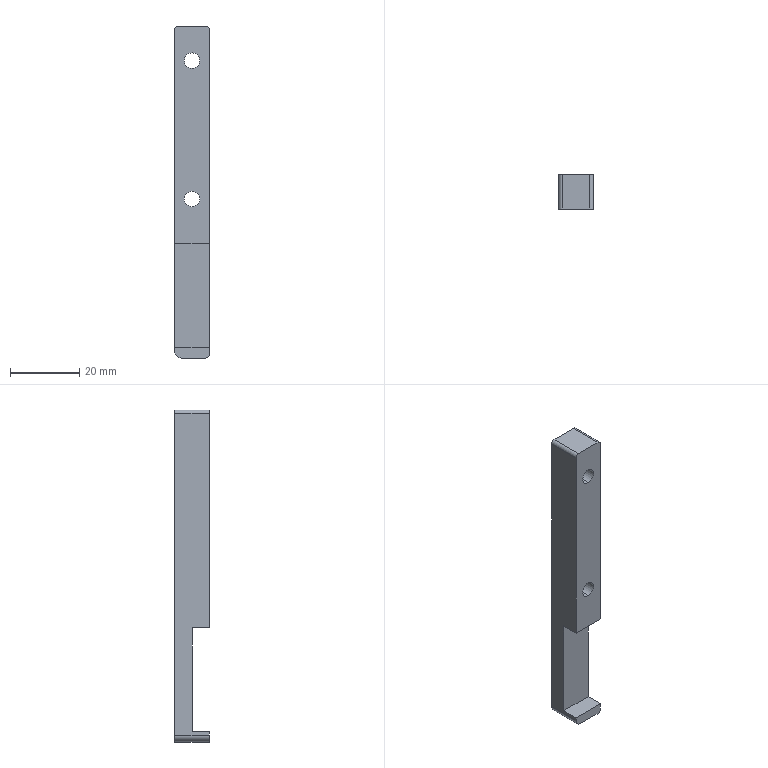Component | SolidWorks | SecondGenerationFour-sidedLabelingFeedingLimitPlate-1 | 1 solid | 24 faces | box 10 x 10 x 96 mm | volume 7451 mm3 | cylinder 12 | plane 12 | commonest cylinder face diameters 8 x4 4.5 x4 2 x3 4 x1
build123d program:
from build123d import *

# Parameters (mm, degrees)
SKETCH1_W                                            = 96
SKETCH1_H                                            = 10
BOSS_EXTRUDE1_DEPTH                                  = 10
HOLE_SIZE_ACCORDING_TO_THE_TYPE_OF_HEXAG_D           = 4.5
HOLE_SIZE_ACCORDING_TO_THE_TYPE_OF_HEXAG_CBORE_D     = 8
HOLE_SIZE_ACCORDING_TO_THE_TYPE_OF_HEXAG_CBORE_DEPTH = 4.6
SKETCH4_W                                            = 30
SKETCH4_H                                            = 5
CUT_EXTRUDE1_DEPTH                                   = 68.974
FILLET1_R                                            = 1
FILLET2_R                                            = 2


with BuildPart() as part:
    # Sketch1 → Boss-Extrude1 (new body)
    with BuildSketch(Plane.XY):
        with Locations((18.487, -24.142)):
            Rectangle(SKETCH1_W, SKETCH1_H)
    extrude(amount=BOSS_EXTRUDE1_DEPTH)

    # Hole Size according to the type of Hexag (through all)
    with Locations(Plane.XY.offset(10)):
        with Locations((-19.513, -24.142), (20.487, -24.142)):
            CounterBoreHole(HOLE_SIZE_ACCORDING_TO_THE_TYPE_OF_HEXAG_D / 2, HOLE_SIZE_ACCORDING_TO_THE_TYPE_OF_HEXAG_CBORE_D / 2, HOLE_SIZE_ACCORDING_TO_THE_TYPE_OF_HEXAG_CBORE_DEPTH)

    # Sketch4 → Cut-Extrude1 (cut, through all)
    with BuildSketch(Plane.XZ.offset(29.142)):
        with Locations((48.487, 2.5)):
            Rectangle(SKETCH4_W, SKETCH4_H)
    extrude(amount=-CUT_EXTRUDE1_DEPTH, mode=Mode.SUBTRACT)

    # Fillet1
    fillet1_edges = [part.edges().sort_by_distance(p)[0] for p in [
        (-29.513, -19.142, 5),
        (66.487, -29.142, 5),
        (-29.513, -29.142, 5),
    ]]
    fillet(fillet1_edges, radius=FILLET1_R)

    # Fillet2
    fillet2_edges = [part.edges().sort_by_distance(p)[0] for p in [
        (66.487, -19.142, 5),
    ]]
    fillet(fillet2_edges, radius=FILLET2_R)


solid = part.part

# Placed as in the assembly
solid = solid.moved(Location((-99.168, 41.863, -153.513), (-90, 0, 90)))
STEP:
#1=CARTESIAN_POINT('',(-2.954,1.861,-5.118));
#2=VERTEX_POINT('',#1);
#3=CARTESIAN_POINT('',(-2.954,1.861,-5.433));
#4=VERTEX_POINT('',#3);
#5=CARTESIAN_POINT('',(-2.954,1.861,-5.276));
#6=DIRECTION('',(0.,1.,0.));
#7=DIRECTION('',(0.,0.,-1.));
#8=AXIS2_PLACEMENT_3D('',#5,#6,#7);
#9=CIRCLE('',#8,0.1575);
#10=EDGE_CURVE('',#2,#4,#9,.T.);
#11=ORIENTED_EDGE('',*,*,#10,.F.);
#12=CARTESIAN_POINT('',(-2.954,2.042,-5.118));
#13=VERTEX_POINT('',#12);
#14=CARTESIAN_POINT('',(-2.954,2.042,-5.118));
#15=DIRECTION('',(0.,1.,0.));
#16=VECTOR('',#15,39.37);
#17=LINE('',#14,#16);
#18=EDGE_CURVE('',#2,#13,#17,.T.);
#19=ORIENTED_EDGE('',*,*,#18,.T.);
#20=CARTESIAN_POINT('',(-2.954,2.042,-5.433));
#21=VERTEX_POINT('',#20);
#22=CARTESIAN_POINT('',(-2.954,2.042,-5.276));
#23=DIRECTION('',(0.,1.,0.));
#24=DIRECTION('',(0.,0.,-1.));
#25=AXIS2_PLACEMENT_3D('',#22,#23,#24);
#26=CIRCLE('',#25,0.1575);
#27=EDGE_CURVE('',#13,#21,#26,.T.);
#28=ORIENTED_EDGE('',*,*,#27,.T.);
#29=CARTESIAN_POINT('',(-2.954,2.042,-5.433));
#30=DIRECTION('',(0.,1.,0.));
#31=VECTOR('',#30,39.37);
#32=LINE('',#29,#31);
#33=EDGE_CURVE('',#4,#21,#32,.T.);
#34=ORIENTED_EDGE('',*,*,#33,.F.);
#35=EDGE_LOOP('',(#11,#19,#28,#34));
#36=FACE_OUTER_BOUND('',#35,.T.);
#37=CARTESIAN_POINT('',(-2.954,2.042,-5.276));
#38=DIRECTION('',(0.,1.,0.));
#39=DIRECTION('',(0.,0.,-1.));
#40=AXIS2_PLACEMENT_3D('',#37,#38,#39);
#41=CYLINDRICAL_SURFACE('',#40,0.1575);
#42=ADVANCED_FACE('',(#36),#41,.F.);
#43=CARTESIAN_POINT('',(-2.954,1.648,-5.187));
#44=VERTEX_POINT('',#43);
#45=CARTESIAN_POINT('',(-2.954,1.648,-5.364));
#46=VERTEX_POINT('',#45);
#47=CARTESIAN_POINT('',(-2.954,1.648,-5.276));
#48=DIRECTION('',(0.,1.,0.));
#49=DIRECTION('',(0.,0.,-1.));
#50=AXIS2_PLACEMENT_3D('',#47,#48,#49);
#51=CIRCLE('',#50,0.08858);
#52=EDGE_CURVE('',#44,#46,#51,.T.);
#53=ORIENTED_EDGE('',*,*,#52,.F.);
#54=CARTESIAN_POINT('',(-2.954,1.861,-5.187));
#55=VERTEX_POINT('',#54);
#56=CARTESIAN_POINT('',(-2.954,2.042,-5.187));
#57=DIRECTION('',(0.,1.,0.));
#58=VECTOR('',#57,39.37);
#59=LINE('',#56,#58);
#60=EDGE_CURVE('',#44,#55,#59,.T.);
#61=ORIENTED_EDGE('',*,*,#60,.T.);
#62=CARTESIAN_POINT('',(-2.954,1.861,-5.364));
#63=VERTEX_POINT('',#62);
#64=CARTESIAN_POINT('',(-2.954,1.861,-5.276));
#65=DIRECTION('',(0.,1.,0.));
#66=DIRECTION('',(0.,0.,-1.));
#67=AXIS2_PLACEMENT_3D('',#64,#65,#66);
#68=CIRCLE('',#67,0.08858);
#69=EDGE_CURVE('',#55,#63,#68,.T.);
#70=ORIENTED_EDGE('',*,*,#69,.T.);
#71=CARTESIAN_POINT('',(-2.954,2.042,-5.364));
#72=DIRECTION('',(0.,1.,0.));
#73=VECTOR('',#72,39.37);
#74=LINE('',#71,#73);
#75=EDGE_CURVE('',#46,#63,#74,.T.);
#76=ORIENTED_EDGE('',*,*,#75,.F.);
#77=EDGE_LOOP('',(#53,#61,#70,#76));
#78=FACE_OUTER_BOUND('',#77,.T.);
#79=CARTESIAN_POINT('',(-2.954,2.042,-5.276));
#80=DIRECTION('',(0.,1.,0.));
#81=DIRECTION('',(0.,0.,-1.));
#82=AXIS2_PLACEMENT_3D('',#79,#80,#81);
#83=CYLINDRICAL_SURFACE('',#82,0.08858);
#84=ADVANCED_FACE('',(#78),#83,.F.);
#85=CARTESIAN_POINT('',(-2.954,1.861,-6.693));
#86=VERTEX_POINT('',#85);
#87=CARTESIAN_POINT('',(-2.954,1.861,-7.008));
#88=VERTEX_POINT('',#87);
#89=CARTESIAN_POINT('',(-2.954,1.861,-6.85));
#90=DIRECTION('',(0.,1.,0.));
#91=DIRECTION('',(0.,0.,-1.));
#92=AXIS2_PLACEMENT_3D('',#89,#90,#91);
#93=CIRCLE('',#92,0.1575);
#94=EDGE_CURVE('',#86,#88,#93,.T.);
#95=ORIENTED_EDGE('',*,*,#94,.F.);
#96=CARTESIAN_POINT('',(-2.954,2.042,-6.693));
#97=VERTEX_POINT('',#96);
#98=CARTESIAN_POINT('',(-2.954,2.042,-6.693));
#99=DIRECTION('',(0.,1.,0.));
#100=VECTOR('',#99,39.37);
#101=LINE('',#98,#100);
#102=EDGE_CURVE('',#86,#97,#101,.T.);
#103=ORIENTED_EDGE('',*,*,#102,.T.);
#104=CARTESIAN_POINT('',(-2.954,2.042,-7.008));
#105=VERTEX_POINT('',#104);
#106=CARTESIAN_POINT('',(-2.954,2.042,-6.85));
#107=DIRECTION('',(0.,1.,0.));
#108=DIRECTION('',(0.,0.,-1.));
#109=AXIS2_PLACEMENT_3D('',#106,#107,#108);
#110=CIRCLE('',#109,0.1575);
#111=EDGE_CURVE('',#97,#105,#110,.T.);
#112=ORIENTED_EDGE('',*,*,#111,.T.);
#113=CARTESIAN_POINT('',(-2.954,2.042,-7.008));
#114=DIRECTION('',(0.,1.,0.));
#115=VECTOR('',#114,39.37);
#116=LINE('',#113,#115);
#117=EDGE_CURVE('',#88,#105,#116,.T.);
#118=ORIENTED_EDGE('',*,*,#117,.F.);
#119=EDGE_LOOP('',(#95,#103,#112,#118));
#120=FACE_OUTER_BOUND('',#119,.T.);
#121=CARTESIAN_POINT('',(-2.954,2.042,-6.85));
#122=DIRECTION('',(0.,1.,0.));
#123=DIRECTION('',(0.,0.,-1.));
#124=AXIS2_PLACEMENT_3D('',#121,#122,#123);
#125=CYLINDRICAL_SURFACE('',#124,0.1575);
#126=ADVANCED_FACE('',(#120),#125,.F.);
#127=CARTESIAN_POINT('',(-2.954,1.648,-6.762));
#128=VERTEX_POINT('',#127);
#129=CARTESIAN_POINT('',(-2.954,1.648,-6.939));
#130=VERTEX_POINT('',#129);
#131=CARTESIAN_POINT('',(-2.954,1.648,-6.85));
#132=DIRECTION('',(0.,1.,0.));
#133=DIRECTION('',(0.,0.,-1.));
#134=AXIS2_PLACEMENT_3D('',#131,#132,#133);
#135=CIRCLE('',#134,0.08858);
#136=EDGE_CURVE('',#128,#130,#135,.T.);
#137=ORIENTED_EDGE('',*,*,#136,.F.);
#138=CARTESIAN_POINT('',(-2.954,1.861,-6.762));
#139=VERTEX_POINT('',#138);
#140=CARTESIAN_POINT('',(-2.954,2.042,-6.762));
#141=DIRECTION('',(0.,1.,0.));
#142=VECTOR('',#141,39.37);
#143=LINE('',#140,#142);
#144=EDGE_CURVE('',#128,#139,#143,.T.);
#145=ORIENTED_EDGE('',*,*,#144,.T.);
#146=CARTESIAN_POINT('',(-2.954,1.861,-6.939));
#147=VERTEX_POINT('',#146);
#148=CARTESIAN_POINT('',(-2.954,1.861,-6.85));
#149=DIRECTION('',(0.,1.,0.));
#150=DIRECTION('',(0.,0.,-1.));
#151=AXIS2_PLACEMENT_3D('',#148,#149,#150);
#152=CIRCLE('',#151,0.08858);
#153=EDGE_CURVE('',#139,#147,#152,.T.);
#154=ORIENTED_EDGE('',*,*,#153,.T.);
#155=CARTESIAN_POINT('',(-2.954,2.042,-6.939));
#156=DIRECTION('',(0.,1.,0.));
#157=VECTOR('',#156,39.37);
#158=LINE('',#155,#157);
#159=EDGE_CURVE('',#130,#147,#158,.T.);
#160=ORIENTED_EDGE('',*,*,#159,.F.);
#161=EDGE_LOOP('',(#137,#145,#154,#160));
#162=FACE_OUTER_BOUND('',#161,.T.);
#163=CARTESIAN_POINT('',(-2.954,2.042,-6.85));
#164=DIRECTION('',(0.,1.,0.));
#165=DIRECTION('',(0.,0.,-1.));
#166=AXIS2_PLACEMENT_3D('',#163,#164,#165);
#167=CYLINDRICAL_SURFACE('',#166,0.08858);
#168=ADVANCED_FACE('',(#162),#167,.F.);
#169=CARTESIAN_POINT('',(-2.954,1.648,-6.85));
#170=DIRECTION('',(0.,1.,0.));
#171=DIRECTION('',(0.,0.,-1.));
#172=AXIS2_PLACEMENT_3D('',#169,#170,#171);
#173=CIRCLE('',#172,0.08858);
#174=EDGE_CURVE('',#130,#128,#173,.T.);
#175=ORIENTED_EDGE('',*,*,#174,.T.);
#176=ORIENTED_EDGE('',*,*,#136,.T.);
#177=EDGE_LOOP('',(#175,#176));
#178=FACE_BOUND('',#177,.T.);
#179=CARTESIAN_POINT('',(-2.954,1.648,-5.276));
#180=DIRECTION('',(0.,1.,0.));
#181=DIRECTION('',(0.,0.,-1.));
#182=AXIS2_PLACEMENT_3D('',#179,#180,#181);
#183=CIRCLE('',#182,0.08858);
#184=EDGE_CURVE('',#46,#44,#183,.T.);
#185=ORIENTED_EDGE('',*,*,#184,.T.);
#186=ORIENTED_EDGE('',*,*,#52,.T.);
#187=EDGE_LOOP('',(#185,#186));
#188=FACE_BOUND('',#187,.T.);
#189=CARTESIAN_POINT('',(-3.111,1.648,-4.882));
#190=VERTEX_POINT('',#189);
#191=CARTESIAN_POINT('',(-2.796,1.648,-4.882));
#192=VERTEX_POINT('',#191);
#193=CARTESIAN_POINT('',(-3.151,1.648,-4.882));
#194=DIRECTION('',(1.,0.,0.));
#195=VECTOR('',#194,39.37);
#196=LINE('',#193,#195);
#197=EDGE_CURVE('',#190,#192,#196,.T.);
#198=ORIENTED_EDGE('',*,*,#197,.F.);
#199=CARTESIAN_POINT('',(-3.151,1.648,-4.921));
#200=VERTEX_POINT('',#199);
#201=CARTESIAN_POINT('',(-3.111,1.648,-4.921));
#202=DIRECTION('',(0.,-1.,0.));
#203=DIRECTION('',(0.,0.,-1.));
#204=AXIS2_PLACEMENT_3D('',#201,#202,#203);
#205=CIRCLE('',#204,0.03937);
#206=EDGE_CURVE('',#190,#200,#205,.T.);
#207=ORIENTED_EDGE('',*,*,#206,.T.);
#208=CARTESIAN_POINT('',(-3.151,1.648,-7.362));
#209=VERTEX_POINT('',#208);
#210=CARTESIAN_POINT('',(-3.151,1.648,-4.882));
#211=DIRECTION('',(0.,0.,1.));
#212=VECTOR('',#211,39.37);
#213=LINE('',#210,#212);
#214=EDGE_CURVE('',#209,#200,#213,.T.);
#215=ORIENTED_EDGE('',*,*,#214,.F.);
#216=CARTESIAN_POINT('',(-2.757,1.648,-7.362));
#217=VERTEX_POINT('',#216);
#218=CARTESIAN_POINT('',(-3.151,1.648,-7.362));
#219=DIRECTION('',(1.,0.,0.));
#220=VECTOR('',#219,39.37);
#221=LINE('',#218,#220);
#222=EDGE_CURVE('',#209,#217,#221,.T.);
#223=ORIENTED_EDGE('',*,*,#222,.T.);
#224=CARTESIAN_POINT('',(-2.757,1.648,-4.921));
#225=VERTEX_POINT('',#224);
#226=CARTESIAN_POINT('',(-2.757,1.648,-4.882));
#227=DIRECTION('',(0.,0.,-1.));
#228=VECTOR('',#227,39.37);
#229=LINE('',#226,#228);
#230=EDGE_CURVE('',#225,#217,#229,.T.);
#231=ORIENTED_EDGE('',*,*,#230,.F.);
#232=CARTESIAN_POINT('',(-2.796,1.648,-4.921));
#233=DIRECTION('',(0.,-1.,0.));
#234=DIRECTION('',(0.,0.,-1.));
#235=AXIS2_PLACEMENT_3D('',#232,#233,#234);
#236=CIRCLE('',#235,0.03937);
#237=EDGE_CURVE('',#225,#192,#236,.T.);
#238=ORIENTED_EDGE('',*,*,#237,.T.);
#239=EDGE_LOOP('',(#198,#207,#215,#223,#231,#238));
#240=FACE_OUTER_BOUND('',#239,.T.);
#241=CARTESIAN_POINT('',(-2.757,1.648,-4.882));
#242=DIRECTION('',(0.,1.,0.));
#243=DIRECTION('',(0.,0.,-1.));
#244=AXIS2_PLACEMENT_3D('',#241,#242,#243);
#245=PLANE('',#244);
#246=ADVANCED_FACE('',(#178,#188,#240),#245,.F.);
#247=CARTESIAN_POINT('',(-3.111,2.042,-4.882));
#248=VERTEX_POINT('',#247);
#249=CARTESIAN_POINT('',(-2.796,2.042,-4.882));
#250=VERTEX_POINT('',#249);
#251=CARTESIAN_POINT('',(-3.151,2.042,-4.882));
#252=DIRECTION('',(1.,0.,0.));
#253=VECTOR('',#252,39.37);
#254=LINE('',#251,#253);
#255=EDGE_CURVE('',#248,#250,#254,.T.);
#256=ORIENTED_EDGE('',*,*,#255,.F.);
#257=CARTESIAN_POINT('',(-3.111,2.042,-4.882));
#258=DIRECTION('',(0.,-1.,0.));
#259=VECTOR('',#258,39.37);
#260=LINE('',#257,#259);
#261=EDGE_CURVE('',#248,#190,#260,.T.);
#262=ORIENTED_EDGE('',*,*,#261,.T.);
#263=ORIENTED_EDGE('',*,*,#197,.T.);
#264=CARTESIAN_POINT('',(-2.796,2.042,-4.882));
#265=DIRECTION('',(0.,1.,0.));
#266=VECTOR('',#265,39.37);
#267=LINE('',#264,#266);
#268=EDGE_CURVE('',#192,#250,#267,.T.);
#269=ORIENTED_EDGE('',*,*,#268,.T.);
#270=EDGE_LOOP('',(#256,#262,#263,#269));
#271=FACE_OUTER_BOUND('',#270,.T.);
#272=CARTESIAN_POINT('',(-3.151,2.042,-4.882));
#273=DIRECTION('',(0.,0.,-1.));
#274=DIRECTION('',(0.,-1.,0.));
#275=AXIS2_PLACEMENT_3D('',#272,#273,#274);
#276=PLANE('',#275);
#277=ADVANCED_FACE('',(#271),#276,.F.);
#278=CARTESIAN_POINT('',(-2.757,1.648,-8.543));
#279=VERTEX_POINT('',#278);
#280=CARTESIAN_POINT('',(-2.757,1.648,-8.622));
#281=VERTEX_POINT('',#280);
#282=CARTESIAN_POINT('',(-2.757,1.648,-4.882));
#283=DIRECTION('',(0.,0.,-1.));
#284=VECTOR('',#283,39.37);
#285=LINE('',#282,#284);
#286=EDGE_CURVE('',#279,#281,#285,.T.);
#287=ORIENTED_EDGE('',*,*,#286,.T.);
#288=CARTESIAN_POINT('',(-2.757,2.042,-8.622));
#289=VERTEX_POINT('',#288);
#290=CARTESIAN_POINT('',(-2.757,2.042,-8.622));
#291=DIRECTION('',(0.,1.,0.));
#292=VECTOR('',#291,39.37);
#293=LINE('',#290,#292);
#294=EDGE_CURVE('',#281,#289,#293,.T.);
#295=ORIENTED_EDGE('',*,*,#294,.T.);
#296=CARTESIAN_POINT('',(-2.757,2.042,-4.921));
#297=VERTEX_POINT('',#296);
#298=CARTESIAN_POINT('',(-2.757,2.042,-4.882));
#299=DIRECTION('',(0.,0.,-1.));
#300=VECTOR('',#299,39.37);
#301=LINE('',#298,#300);
#302=EDGE_CURVE('',#297,#289,#301,.T.);
#303=ORIENTED_EDGE('',*,*,#302,.F.);
#304=CARTESIAN_POINT('',(-2.757,2.042,-4.921));
#305=DIRECTION('',(0.,-1.,0.));
#306=VECTOR('',#305,39.37);
#307=LINE('',#304,#306);
#308=EDGE_CURVE('',#297,#225,#307,.T.);
#309=ORIENTED_EDGE('',*,*,#308,.T.);
#310=ORIENTED_EDGE('',*,*,#230,.T.);
#311=CARTESIAN_POINT('',(-2.757,1.845,-7.362));
#312=VERTEX_POINT('',#311);
#313=CARTESIAN_POINT('',(-2.757,1.845,-7.362));
#314=DIRECTION('',(0.,-1.,0.));
#315=VECTOR('',#314,39.37);
#316=LINE('',#313,#315);
#317=EDGE_CURVE('',#312,#217,#316,.T.);
#318=ORIENTED_EDGE('',*,*,#317,.F.);
#319=CARTESIAN_POINT('',(-2.757,1.845,-8.543));
#320=VERTEX_POINT('',#319);
#321=CARTESIAN_POINT('',(-2.757,1.845,-7.362));
#322=DIRECTION('',(0.,0.,1.));
#323=VECTOR('',#322,39.37);
#324=LINE('',#321,#323);
#325=EDGE_CURVE('',#320,#312,#324,.T.);
#326=ORIENTED_EDGE('',*,*,#325,.F.);
#327=CARTESIAN_POINT('',(-2.757,1.845,-8.543));
#328=DIRECTION('',(0.,1.,0.));
#329=VECTOR('',#328,39.37);
#330=LINE('',#327,#329);
#331=EDGE_CURVE('',#279,#320,#330,.T.);
#332=ORIENTED_EDGE('',*,*,#331,.F.);
#333=EDGE_LOOP('',(#287,#295,#303,#309,#310,#318,#326,#332));
#334=FACE_OUTER_BOUND('',#333,.T.);
#335=CARTESIAN_POINT('',(-2.757,2.042,-4.882));
#336=DIRECTION('',(-1.,0.,0.));
#337=DIRECTION('',(0.,1.,0.));
#338=AXIS2_PLACEMENT_3D('',#335,#336,#337);
#339=PLANE('',#338);
#340=ADVANCED_FACE('',(#334),#339,.F.);
#341=CARTESIAN_POINT('',(-2.796,1.648,-8.661));
#342=VERTEX_POINT('',#341);
#343=CARTESIAN_POINT('',(-3.072,1.648,-8.661));
#344=VERTEX_POINT('',#343);
#345=CARTESIAN_POINT('',(-3.151,1.648,-8.661));
#346=DIRECTION('',(-1.,0.,0.));
#347=VECTOR('',#346,39.37);
#348=LINE('',#345,#347);
#349=EDGE_CURVE('',#342,#344,#348,.T.);
#350=ORIENTED_EDGE('',*,*,#349,.T.);
#351=CARTESIAN_POINT('',(-3.072,2.042,-8.661));
#352=VERTEX_POINT('',#351);
#353=CARTESIAN_POINT('',(-3.072,2.042,-8.661));
#354=DIRECTION('',(0.,1.,0.));
#355=VECTOR('',#354,39.37);
#356=LINE('',#353,#355);
#357=EDGE_CURVE('',#344,#352,#356,.T.);
#358=ORIENTED_EDGE('',*,*,#357,.T.);
#359=CARTESIAN_POINT('',(-2.796,2.042,-8.661));
#360=VERTEX_POINT('',#359);
#361=CARTESIAN_POINT('',(-3.151,2.042,-8.661));
#362=DIRECTION('',(-1.,0.,0.));
#363=VECTOR('',#362,39.37);
#364=LINE('',#361,#363);
#365=EDGE_CURVE('',#360,#352,#364,.T.);
#366=ORIENTED_EDGE('',*,*,#365,.F.);
#367=CARTESIAN_POINT('',(-2.796,2.042,-8.661));
#368=DIRECTION('',(0.,-1.,0.));
#369=VECTOR('',#368,39.37);
#370=LINE('',#367,#369);
#371=EDGE_CURVE('',#360,#342,#370,.T.);
#372=ORIENTED_EDGE('',*,*,#371,.T.);
#373=EDGE_LOOP('',(#350,#358,#366,#372));
#374=FACE_OUTER_BOUND('',#373,.T.);
#375=CARTESIAN_POINT('',(-3.151,2.042,-8.661));
#376=DIRECTION('',(0.,0.,1.));
#377=DIRECTION('',(0.,1.,0.));
#378=AXIS2_PLACEMENT_3D('',#375,#376,#377);
#379=PLANE('',#378);
#380=ADVANCED_FACE('',(#374),#379,.F.);
#381=CARTESIAN_POINT('',(-3.151,2.042,-8.583));
#382=VERTEX_POINT('',#381);
#383=CARTESIAN_POINT('',(-3.151,2.042,-4.921));
#384=VERTEX_POINT('',#383);
#385=CARTESIAN_POINT('',(-3.151,2.042,-4.882));
#386=DIRECTION('',(0.,0.,1.));
#387=VECTOR('',#386,39.37);
#388=LINE('',#385,#387);
#389=EDGE_CURVE('',#382,#384,#388,.T.);
#390=ORIENTED_EDGE('',*,*,#389,.F.);
#391=CARTESIAN_POINT('',(-3.151,1.648,-8.583));
#392=VERTEX_POINT('',#391);
#393=CARTESIAN_POINT('',(-3.151,2.042,-8.583));
#394=DIRECTION('',(0.,-1.,0.));
#395=VECTOR('',#394,39.37);
#396=LINE('',#393,#395);
#397=EDGE_CURVE('',#382,#392,#396,.T.);
#398=ORIENTED_EDGE('',*,*,#397,.T.);
#399=CARTESIAN_POINT('',(-3.151,1.648,-8.543));
#400=VERTEX_POINT('',#399);
#401=CARTESIAN_POINT('',(-3.151,1.648,-4.882));
#402=DIRECTION('',(0.,0.,1.));
#403=VECTOR('',#402,39.37);
#404=LINE('',#401,#403);
#405=EDGE_CURVE('',#392,#400,#404,.T.);
#406=ORIENTED_EDGE('',*,*,#405,.T.);
#407=CARTESIAN_POINT('',(-3.151,1.845,-8.543));
#408=VERTEX_POINT('',#407);
#409=CARTESIAN_POINT('',(-3.151,1.845,-8.543));
#410=DIRECTION('',(0.,1.,0.));
#411=VECTOR('',#410,39.37);
#412=LINE('',#409,#411);
#413=EDGE_CURVE('',#400,#408,#412,.T.);
#414=ORIENTED_EDGE('',*,*,#413,.T.);
#415=CARTESIAN_POINT('',(-3.151,1.845,-7.362));
#416=VERTEX_POINT('',#415);
#417=CARTESIAN_POINT('',(-3.151,1.845,-7.362));
#418=DIRECTION('',(0.,0.,1.));
#419=VECTOR('',#418,39.37);
#420=LINE('',#417,#419);
#421=EDGE_CURVE('',#408,#416,#420,.T.);
#422=ORIENTED_EDGE('',*,*,#421,.T.);
#423=CARTESIAN_POINT('',(-3.151,1.845,-7.362));
#424=DIRECTION('',(0.,-1.,0.));
#425=VECTOR('',#424,39.37);
#426=LINE('',#423,#425);
#427=EDGE_CURVE('',#416,#209,#426,.T.);
#428=ORIENTED_EDGE('',*,*,#427,.T.);
#429=ORIENTED_EDGE('',*,*,#214,.T.);
#430=CARTESIAN_POINT('',(-3.151,2.042,-4.921));
#431=DIRECTION('',(0.,1.,0.));
#432=VECTOR('',#431,39.37);
#433=LINE('',#430,#432);
#434=EDGE_CURVE('',#200,#384,#433,.T.);
#435=ORIENTED_EDGE('',*,*,#434,.T.);
#436=EDGE_LOOP('',(#390,#398,#406,#414,#422,#428,#429,#435));
#437=FACE_OUTER_BOUND('',#436,.T.);
#438=CARTESIAN_POINT('',(-3.151,2.042,-4.882));
#439=DIRECTION('',(1.,0.,0.));
#440=DIRECTION('',(0.,-1.,0.));
#441=AXIS2_PLACEMENT_3D('',#438,#439,#440);
#442=PLANE('',#441);
#443=ADVANCED_FACE('',(#437),#442,.F.);
#444=CARTESIAN_POINT('',(-2.954,2.042,-5.276));
#445=DIRECTION('',(0.,1.,0.));
#446=DIRECTION('',(0.,0.,-1.));
#447=AXIS2_PLACEMENT_3D('',#444,#445,#446);
#448=CIRCLE('',#447,0.1575);
#449=EDGE_CURVE('',#21,#13,#448,.T.);
#450=ORIENTED_EDGE('',*,*,#449,.F.);
#451=ORIENTED_EDGE('',*,*,#27,.F.);
#452=EDGE_LOOP('',(#450,#451));
#453=FACE_BOUND('',#452,.T.);
#454=CARTESIAN_POINT('',(-2.954,2.042,-6.85));
#455=DIRECTION('',(0.,1.,0.));
#456=DIRECTION('',(0.,0.,-1.));
#457=AXIS2_PLACEMENT_3D('',#454,#455,#456);
#458=CIRCLE('',#457,0.1575);
#459=EDGE_CURVE('',#105,#97,#458,.T.);
#460=ORIENTED_EDGE('',*,*,#459,.F.);
#461=ORIENTED_EDGE('',*,*,#111,.F.);
#462=EDGE_LOOP('',(#460,#461));
#463=FACE_BOUND('',#462,.T.);
#464=ORIENTED_EDGE('',*,*,#365,.T.);
#465=CARTESIAN_POINT('',(-3.072,2.042,-8.583));
#466=DIRECTION('',(0.,1.,0.));
#467=DIRECTION('',(0.,0.,-1.));
#468=AXIS2_PLACEMENT_3D('',#465,#466,#467);
#469=CIRCLE('',#468,0.07874);
#470=EDGE_CURVE('',#352,#382,#469,.T.);
#471=ORIENTED_EDGE('',*,*,#470,.T.);
#472=ORIENTED_EDGE('',*,*,#389,.T.);
#473=CARTESIAN_POINT('',(-3.111,2.042,-4.921));
#474=DIRECTION('',(0.,1.,0.));
#475=DIRECTION('',(0.,0.,-1.));
#476=AXIS2_PLACEMENT_3D('',#473,#474,#475);
#477=CIRCLE('',#476,0.03937);
#478=EDGE_CURVE('',#384,#248,#477,.T.);
#479=ORIENTED_EDGE('',*,*,#478,.T.);
#480=ORIENTED_EDGE('',*,*,#255,.T.);
#481=CARTESIAN_POINT('',(-2.796,2.042,-4.921));
#482=DIRECTION('',(0.,1.,0.));
#483=DIRECTION('',(0.,0.,-1.));
#484=AXIS2_PLACEMENT_3D('',#481,#482,#483);
#485=CIRCLE('',#484,0.03937);
#486=EDGE_CURVE('',#250,#297,#485,.T.);
#487=ORIENTED_EDGE('',*,*,#486,.T.);
#488=ORIENTED_EDGE('',*,*,#302,.T.);
#489=CARTESIAN_POINT('',(-2.796,2.042,-8.622));
#490=DIRECTION('',(0.,1.,0.));
#491=DIRECTION('',(0.,0.,-1.));
#492=AXIS2_PLACEMENT_3D('',#489,#490,#491);
#493=CIRCLE('',#492,0.03937);
#494=EDGE_CURVE('',#289,#360,#493,.T.);
#495=ORIENTED_EDGE('',*,*,#494,.T.);
#496=EDGE_LOOP('',(#464,#471,#472,#479,#480,#487,#488,#495));
#497=FACE_OUTER_BOUND('',#496,.T.);
#498=CARTESIAN_POINT('',(-2.757,2.042,-4.882));
#499=DIRECTION('',(0.,1.,0.));
#500=DIRECTION('',(0.,0.,-1.));
#501=AXIS2_PLACEMENT_3D('',#498,#499,#500);
#502=PLANE('',#501);
#503=ADVANCED_FACE('',(#453,#463,#497),#502,.T.);
#504=ORIENTED_EDGE('',*,*,#405,.F.);
#505=CARTESIAN_POINT('',(-3.072,1.648,-8.583));
#506=DIRECTION('',(0.,-1.,0.));
#507=DIRECTION('',(0.,0.,-1.));
#508=AXIS2_PLACEMENT_3D('',#505,#506,#507);
#509=CIRCLE('',#508,0.07874);
#510=EDGE_CURVE('',#392,#344,#509,.T.);
#511=ORIENTED_EDGE('',*,*,#510,.T.);
#512=ORIENTED_EDGE('',*,*,#349,.F.);
#513=CARTESIAN_POINT('',(-2.796,1.648,-8.622));
#514=DIRECTION('',(0.,-1.,0.));
#515=DIRECTION('',(0.,0.,-1.));
#516=AXIS2_PLACEMENT_3D('',#513,#514,#515);
#517=CIRCLE('',#516,0.03937);
#518=EDGE_CURVE('',#342,#281,#517,.T.);
#519=ORIENTED_EDGE('',*,*,#518,.T.);
#520=ORIENTED_EDGE('',*,*,#286,.F.);
#521=CARTESIAN_POINT('',(-3.151,1.648,-8.543));
#522=DIRECTION('',(1.,0.,0.));
#523=VECTOR('',#522,39.37);
#524=LINE('',#521,#523);
#525=EDGE_CURVE('',#400,#279,#524,.T.);
#526=ORIENTED_EDGE('',*,*,#525,.F.);
#527=EDGE_LOOP('',(#504,#511,#512,#519,#520,#526));
#528=FACE_OUTER_BOUND('',#527,.T.);
#529=CARTESIAN_POINT('',(-2.757,1.648,-4.882));
#530=DIRECTION('',(0.,1.,0.));
#531=DIRECTION('',(0.,0.,-1.));
#532=AXIS2_PLACEMENT_3D('',#529,#530,#531);
#533=PLANE('',#532);
#534=ADVANCED_FACE('',(#528),#533,.F.);
#535=ORIENTED_EDGE('',*,*,#144,.F.);
#536=ORIENTED_EDGE('',*,*,#174,.F.);
#537=ORIENTED_EDGE('',*,*,#159,.T.);
#538=CARTESIAN_POINT('',(-2.954,1.861,-6.85));
#539=DIRECTION('',(0.,1.,0.));
#540=DIRECTION('',(0.,0.,-1.));
#541=AXIS2_PLACEMENT_3D('',#538,#539,#540);
#542=CIRCLE('',#541,0.08858);
#543=EDGE_CURVE('',#147,#139,#542,.T.);
#544=ORIENTED_EDGE('',*,*,#543,.T.);
#545=EDGE_LOOP('',(#535,#536,#537,#544));
#546=FACE_OUTER_BOUND('',#545,.T.);
#547=CARTESIAN_POINT('',(-2.954,2.042,-6.85));
#548=DIRECTION('',(0.,1.,0.));
#549=DIRECTION('',(0.,0.,-1.));
#550=AXIS2_PLACEMENT_3D('',#547,#548,#549);
#551=CYLINDRICAL_SURFACE('',#550,0.08858);
#552=ADVANCED_FACE('',(#546),#551,.F.);
#553=ORIENTED_EDGE('',*,*,#543,.F.);
#554=ORIENTED_EDGE('',*,*,#153,.F.);
#555=EDGE_LOOP('',(#553,#554));
#556=FACE_BOUND('',#555,.T.);
#557=CARTESIAN_POINT('',(-2.954,1.861,-6.85));
#558=DIRECTION('',(0.,1.,0.));
#559=DIRECTION('',(0.,0.,-1.));
#560=AXIS2_PLACEMENT_3D('',#557,#558,#559);
#561=CIRCLE('',#560,0.1575);
#562=EDGE_CURVE('',#88,#86,#561,.T.);
#563=ORIENTED_EDGE('',*,*,#562,.T.);
#564=ORIENTED_EDGE('',*,*,#94,.T.);
#565=EDGE_LOOP('',(#563,#564));
#566=FACE_OUTER_BOUND('',#565,.T.);
#567=CARTESIAN_POINT('',(-2.954,1.861,-6.939));
#568=DIRECTION('',(0.,-1.,0.));
#569=DIRECTION('',(0.,0.,1.));
#570=AXIS2_PLACEMENT_3D('',#567,#568,#569);
#571=PLANE('',#570);
#572=ADVANCED_FACE('',(#556,#566),#571,.F.);
#573=ORIENTED_EDGE('',*,*,#102,.F.);
#574=ORIENTED_EDGE('',*,*,#562,.F.);
#575=ORIENTED_EDGE('',*,*,#117,.T.);
#576=ORIENTED_EDGE('',*,*,#459,.T.);
#577=EDGE_LOOP('',(#573,#574,#575,#576));
#578=FACE_OUTER_BOUND('',#577,.T.);
#579=CARTESIAN_POINT('',(-2.954,2.042,-6.85));
#580=DIRECTION('',(0.,1.,0.));
#581=DIRECTION('',(0.,0.,-1.));
#582=AXIS2_PLACEMENT_3D('',#579,#580,#581);
#583=CYLINDRICAL_SURFACE('',#582,0.1575);
#584=ADVANCED_FACE('',(#578),#583,.F.);
#585=ORIENTED_EDGE('',*,*,#60,.F.);
#586=ORIENTED_EDGE('',*,*,#184,.F.);
#587=ORIENTED_EDGE('',*,*,#75,.T.);
#588=CARTESIAN_POINT('',(-2.954,1.861,-5.276));
#589=DIRECTION('',(0.,1.,0.));
#590=DIRECTION('',(0.,0.,-1.));
#591=AXIS2_PLACEMENT_3D('',#588,#589,#590);
#592=CIRCLE('',#591,0.08858);
#593=EDGE_CURVE('',#63,#55,#592,.T.);
#594=ORIENTED_EDGE('',*,*,#593,.T.);
#595=EDGE_LOOP('',(#585,#586,#587,#594));
#596=FACE_OUTER_BOUND('',#595,.T.);
#597=CARTESIAN_POINT('',(-2.954,2.042,-5.276));
#598=DIRECTION('',(0.,1.,0.));
#599=DIRECTION('',(0.,0.,-1.));
#600=AXIS2_PLACEMENT_3D('',#597,#598,#599);
#601=CYLINDRICAL_SURFACE('',#600,0.08858);
#602=ADVANCED_FACE('',(#596),#601,.F.);
#603=ORIENTED_EDGE('',*,*,#593,.F.);
#604=ORIENTED_EDGE('',*,*,#69,.F.);
#605=EDGE_LOOP('',(#603,#604));
#606=FACE_BOUND('',#605,.T.);
#607=CARTESIAN_POINT('',(-2.954,1.861,-5.276));
#608=DIRECTION('',(0.,1.,0.));
#609=DIRECTION('',(0.,0.,-1.));
#610=AXIS2_PLACEMENT_3D('',#607,#608,#609);
#611=CIRCLE('',#610,0.1575);
#612=EDGE_CURVE('',#4,#2,#611,.T.);
#613=ORIENTED_EDGE('',*,*,#612,.T.);
#614=ORIENTED_EDGE('',*,*,#10,.T.);
#615=EDGE_LOOP('',(#613,#614));
#616=FACE_OUTER_BOUND('',#615,.T.);
#617=CARTESIAN_POINT('',(-2.954,1.861,-5.364));
#618=DIRECTION('',(0.,-1.,0.));
#619=DIRECTION('',(0.,0.,1.));
#620=AXIS2_PLACEMENT_3D('',#617,#618,#619);
#621=PLANE('',#620);
#622=ADVANCED_FACE('',(#606,#616),#621,.F.);
#623=ORIENTED_EDGE('',*,*,#18,.F.);
#624=ORIENTED_EDGE('',*,*,#612,.F.);
#625=ORIENTED_EDGE('',*,*,#33,.T.);
#626=ORIENTED_EDGE('',*,*,#449,.T.);
#627=EDGE_LOOP('',(#623,#624,#625,#626));
#628=FACE_OUTER_BOUND('',#627,.T.);
#629=CARTESIAN_POINT('',(-2.954,2.042,-5.276));
#630=DIRECTION('',(0.,1.,0.));
#631=DIRECTION('',(0.,0.,-1.));
#632=AXIS2_PLACEMENT_3D('',#629,#630,#631);
#633=CYLINDRICAL_SURFACE('',#632,0.1575);
#634=ADVANCED_FACE('',(#628),#633,.F.);
#635=ORIENTED_EDGE('',*,*,#317,.T.);
#636=ORIENTED_EDGE('',*,*,#222,.F.);
#637=ORIENTED_EDGE('',*,*,#427,.F.);
#638=CARTESIAN_POINT('',(-3.151,1.845,-7.362));
#639=DIRECTION('',(1.,0.,0.));
#640=VECTOR('',#639,39.37);
#641=LINE('',#638,#640);
#642=EDGE_CURVE('',#416,#312,#641,.T.);
#643=ORIENTED_EDGE('',*,*,#642,.T.);
#644=EDGE_LOOP('',(#635,#636,#637,#643));
#645=FACE_OUTER_BOUND('',#644,.T.);
#646=CARTESIAN_POINT('',(-3.151,1.845,-7.362));
#647=DIRECTION('',(0.,0.,1.));
#648=DIRECTION('',(0.,1.,0.));
#649=AXIS2_PLACEMENT_3D('',#646,#647,#648);
#650=PLANE('',#649);
#651=ADVANCED_FACE('',(#645),#650,.F.);
#652=ORIENTED_EDGE('',*,*,#325,.T.);
#653=ORIENTED_EDGE('',*,*,#642,.F.);
#654=ORIENTED_EDGE('',*,*,#421,.F.);
#655=CARTESIAN_POINT('',(-3.151,1.845,-8.543));
#656=DIRECTION('',(1.,0.,0.));
#657=VECTOR('',#656,39.37);
#658=LINE('',#655,#657);
#659=EDGE_CURVE('',#408,#320,#658,.T.);
#660=ORIENTED_EDGE('',*,*,#659,.T.);
#661=EDGE_LOOP('',(#652,#653,#654,#660));
#662=FACE_OUTER_BOUND('',#661,.T.);
#663=CARTESIAN_POINT('',(-3.151,1.845,-7.362));
#664=DIRECTION('',(0.,1.,0.));
#665=DIRECTION('',(0.,0.,-1.));
#666=AXIS2_PLACEMENT_3D('',#663,#664,#665);
#667=PLANE('',#666);
#668=ADVANCED_FACE('',(#662),#667,.F.);
#669=ORIENTED_EDGE('',*,*,#331,.T.);
#670=ORIENTED_EDGE('',*,*,#659,.F.);
#671=ORIENTED_EDGE('',*,*,#413,.F.);
#672=ORIENTED_EDGE('',*,*,#525,.T.);
#673=EDGE_LOOP('',(#669,#670,#671,#672));
#674=FACE_OUTER_BOUND('',#673,.T.);
#675=CARTESIAN_POINT('',(-3.151,1.845,-8.543));
#676=DIRECTION('',(0.,0.,-1.));
#677=DIRECTION('',(0.,-1.,0.));
#678=AXIS2_PLACEMENT_3D('',#675,#676,#677);
#679=PLANE('',#678);
#680=ADVANCED_FACE('',(#674),#679,.F.);
#681=ORIENTED_EDGE('',*,*,#478,.F.);
#682=ORIENTED_EDGE('',*,*,#434,.F.);
#683=ORIENTED_EDGE('',*,*,#206,.F.);
#684=ORIENTED_EDGE('',*,*,#261,.F.);
#685=EDGE_LOOP('',(#681,#682,#683,#684));
#686=FACE_OUTER_BOUND('',#685,.T.);
#687=CARTESIAN_POINT('',(-3.111,2.042,-4.921));
#688=DIRECTION('',(0.,-1.,0.));
#689=DIRECTION('',(0.,0.,1.));
#690=AXIS2_PLACEMENT_3D('',#687,#688,#689);
#691=CYLINDRICAL_SURFACE('',#690,0.03937);
#692=ADVANCED_FACE('',(#686),#691,.T.);
#693=ORIENTED_EDGE('',*,*,#494,.F.);
#694=ORIENTED_EDGE('',*,*,#294,.F.);
#695=ORIENTED_EDGE('',*,*,#518,.F.);
#696=ORIENTED_EDGE('',*,*,#371,.F.);
#697=EDGE_LOOP('',(#693,#694,#695,#696));
#698=FACE_OUTER_BOUND('',#697,.T.);
#699=CARTESIAN_POINT('',(-2.796,2.042,-8.622));
#700=DIRECTION('',(0.,-1.,0.));
#701=DIRECTION('',(0.,0.,1.));
#702=AXIS2_PLACEMENT_3D('',#699,#700,#701);
#703=CYLINDRICAL_SURFACE('',#702,0.03937);
#704=ADVANCED_FACE('',(#698),#703,.T.);
#705=ORIENTED_EDGE('',*,*,#486,.F.);
#706=ORIENTED_EDGE('',*,*,#268,.F.);
#707=ORIENTED_EDGE('',*,*,#237,.F.);
#708=ORIENTED_EDGE('',*,*,#308,.F.);
#709=EDGE_LOOP('',(#705,#706,#707,#708));
#710=FACE_OUTER_BOUND('',#709,.T.);
#711=CARTESIAN_POINT('',(-2.796,2.042,-4.921));
#712=DIRECTION('',(0.,-1.,0.));
#713=DIRECTION('',(0.,0.,1.));
#714=AXIS2_PLACEMENT_3D('',#711,#712,#713);
#715=CYLINDRICAL_SURFACE('',#714,0.03937);
#716=ADVANCED_FACE('',(#710),#715,.T.);
#717=ORIENTED_EDGE('',*,*,#470,.F.);
#718=ORIENTED_EDGE('',*,*,#357,.F.);
#719=ORIENTED_EDGE('',*,*,#510,.F.);
#720=ORIENTED_EDGE('',*,*,#397,.F.);
#721=EDGE_LOOP('',(#717,#718,#719,#720));
#722=FACE_OUTER_BOUND('',#721,.T.);
#723=CARTESIAN_POINT('',(-3.072,2.042,-8.583));
#724=DIRECTION('',(0.,-1.,0.));
#725=DIRECTION('',(0.,0.,1.));
#726=AXIS2_PLACEMENT_3D('',#723,#724,#725);
#727=CYLINDRICAL_SURFACE('',#726,0.07874);
#728=ADVANCED_FACE('',(#722),#727,.T.);
#729=CLOSED_SHELL('',(#42,#84,#126,#168,#246,#277,#340,#380,#443,#503,#534,#552,#572,#584,#602,#622,#634,#651,#668,#680,#692,#704,#716,#728));
#730=MANIFOLD_SOLID_BREP('',#729);
#731=CARTESIAN_POINT('',(0.,0.,0.));
#732=DIRECTION('',(0.,0.,1.));
#733=DIRECTION('',(1.,0.,0.));
#734=AXIS2_PLACEMENT_3D('',#731,#732,#733);
#735=(LENGTH_UNIT()NAMED_UNIT(*)SI_UNIT($,.METRE.));
#736=LENGTH_MEASURE_WITH_UNIT(LENGTH_MEASURE(0.0254),#735);
#737=DIMENSIONAL_EXPONENTS(1.,0.,0.,0.,0.,0.,0.);
#738=(CONVERSION_BASED_UNIT('',#736)LENGTH_UNIT()NAMED_UNIT(#737));
#739=UNCERTAINTY_MEASURE_WITH_UNIT(LENGTH_MEASURE(0.00001),#738,'','');
#740=(NAMED_UNIT(*)PLANE_ANGLE_UNIT()SI_UNIT($,.RADIAN.));
#741=(NAMED_UNIT(*)SI_UNIT($,.STERADIAN.)SOLID_ANGLE_UNIT());
#742=(GEOMETRIC_REPRESENTATION_CONTEXT(3)GLOBAL_UNCERTAINTY_ASSIGNED_CONTEXT((#739))GLOBAL_UNIT_ASSIGNED_CONTEXT((#738,#740,#741))REPRESENTATION_CONTEXT('',''));
#743=ADVANCED_BREP_SHAPE_REPRESENTATION('',(#730,#734),#742);
#744=COLOUR_RGB('',0.7922,0.8196,0.9333);
#745=FILL_AREA_STYLE_COLOUR('',#744);
#746=FILL_AREA_STYLE('',(#745));
#747=SURFACE_STYLE_FILL_AREA(#746);
#748=SURFACE_SIDE_STYLE('',(#747));
#749=SURFACE_STYLE_USAGE(.BOTH.,#748);
#750=PRESENTATION_STYLE_ASSIGNMENT((#749));
#751=STYLED_ITEM('',(#750),#730);
#752=PRESENTATION_LAYER_ASSIGNMENT('','',(#751));
#753=(LENGTH_UNIT()NAMED_UNIT(*)SI_UNIT($,.METRE.));
#754=LENGTH_MEASURE_WITH_UNIT(LENGTH_MEASURE(0.0254),#753);
#755=DIMENSIONAL_EXPONENTS(1.,0.,0.,0.,0.,0.,0.);
#756=(CONVERSION_BASED_UNIT('',#754)LENGTH_UNIT()NAMED_UNIT(#755));
#757=UNCERTAINTY_MEASURE_WITH_UNIT(LENGTH_MEASURE(0.00001),#756,'','');
#758=(NAMED_UNIT(*)PLANE_ANGLE_UNIT()SI_UNIT($,.RADIAN.));
#759=(NAMED_UNIT(*)SI_UNIT($,.STERADIAN.)SOLID_ANGLE_UNIT());
#760=(GEOMETRIC_REPRESENTATION_CONTEXT(3)GLOBAL_UNCERTAINTY_ASSIGNED_CONTEXT((#757))GLOBAL_UNIT_ASSIGNED_CONTEXT((#756,#758,#759))REPRESENTATION_CONTEXT('',''));
#761=MECHANICAL_DESIGN_GEOMETRIC_PRESENTATION_REPRESENTATION('',(#751),#760);